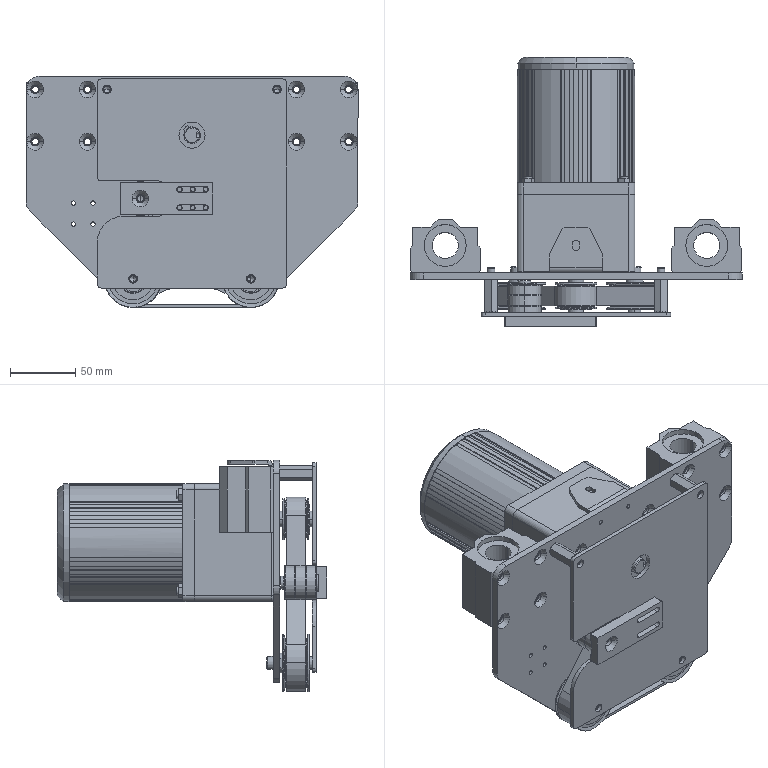Assembly | SolidWorks | mm | 19 component files | 21 solids | 2403 faces | box 254 x 206 x 177 mm | volume 1642860 mm3 | cylinder 1465 | plane 415 | cone 335 | torus 188 | commonest cylinder face diameters 0.56 x272 0.3 x253 3.95 x244 35.22 x82 37.44 x80 6.6 x38 25.67 x32 27.89 x31
Bill of materials:
BAY6000ZZ-J.stp | 3 | AISI 304 | Short thick annular ring with a central through bore; the face shows concentric outer ring, a recessed annular band, and an inner ring, like a shielded ball bearing seen from outside.
Belt11 | 1 |  | Thin-walled closed loop band of constant width. Its outline is a rounded, roughly triangular shape with an inward bend on one side.
EBF41-S3M150-30-A-N-d12.stp | 1 | 6061 Alloy | Toothed pulley-like cylinder with flanges at both ends and short hub bosses, a central bore with a keyway, and radial holes through the toothed rim.
EVD21-40-S3M150.stp | 2 | 6061 Alloy | Toothed pulley-like cylinder with flanges at both ends, a raised annular hub face on each side, and a plain central through bore with no keyway.
IK-AC(40W)InductionMotor[5IK40A1-C] | 1 |  | Square box-shaped block with rounded edges, joined coaxially to a longer cylindrical body that has lengthwise grooves and a chamfered far end. A single shaft sticks out of the square front face, off-centre, from a short stepped round boss. The overall form looks like a geared motor, but this is only a guess from the shape.
LMW01-d20.stp | 2 | 6061 Alloy | Prismatic housing block with a large through bore. The profile is stepped, with a raised top boss and stepped, chamfered lower shoulders. Four small holes are on one face, and there is an annular recess around the bore on the top face.
MDJ12-10-Y2-F23-E10-N6.stp | 2 | 45 | Stepped cylindrical pin. It has a long plain shank, a collar flange with two parallel flats, a narrow neck groove, and a short chamfered end section. An axial hole with a conical bottom is at one end.
MED02-10-Y2-F24.stp | 1 | 45 | Flanged cylindrical bushing/pin. It has a flange with two flats at one end, a long cylindrical body, a shallow circumferential groove near the opposite end, and an axial bore.
QX1-03-BJMotorMountingPlate | 1 | 201 Annealed Stainless Steel (SS) | Flat plate with a rectangular upper portion and tapered lower sides ending in a concave arc cutout. It has a large central round hole and many smaller holes, some with chamfered or countersunk edges.
QX1-08-BJAdapterBracket | 1 | Q235 | L-shaped bent plate bracket. One leg is tapered with a single elongated slot. The other leg is rectangular with two round holes. The two legs meet at a radiused bend.
QX1-23-BJCoverPlate | 1 | Q235 | Thin, nearly square flat plate with a rectangular notch cut into one side. It has a large round hole, a 2x3 grid of small holes, and four mounting holes near the corners.
QX1-24-TensionerSeat | 1 | 6061 Alloy | Rectangular bar with small chamfered corners. It has one countersunk through hole near one end and two parallel obround slots near the other end.
RBE12-S10-L25-M6-N6.stp | 2 |  | Hexagonal standoff-like part. It has a hex body with a female axial bore at one end, and a smaller cylindrical male stud with a relief neck and chamfered tip at the other.
Mates:
1. coincident | QX1-03-BJMotorMountingPlate-1 face at (52.203, 5.084, 478.747) dir (0, 1, 0) | IK-AC(40W)InductionMotor[5IK40A1-C]-1 face at (97.203, 5.084, 545.747) dir (0, -1, 0)
2. concentric | QX1-03-BJMotorMountingPlate-1 face at (52.203, 5.084, 518.747) dir (0, -1, 0) r 17.15 | IK-AC(40W)InductionMotor[5IK40A1-C]-1 face at (52.203, 5.084, 518.747) dir (0, 1, 0) r 6
3. parallel | QX1-03-BJMotorMountingPlate-1 face at (-74.797, 5.084, 563.747) dir (0, 0, 1) | IK-AC(40W)InductionMotor[5IK40A1-C]-1 face at (97.203, 65.084, 545.747) dir (0, 0, 1)
4. concentric | QX1-03-BJMotorMountingPlate-1 face at (7.203, 5.084, 408.747) dir (0, -1, 0) r 5.25 | EVD21-40-S3M150.stp-1 face at (7.203, -7.916, 408.747) dir (0, 1, 0) r 5
5. concentric | QX1-03-BJMotorMountingPlate-1 face at (97.203, 5.084, 408.747) dir (0, -1, 0) r 5.25 | EVD21-40-S3M150.stp-2 face at (97.203, -7.916, 408.747) dir (0, 1, 0) r 5
6. coincident | QX1-03-BJMotorMountingPlate-1 face at (52.203, 5.084, 478.747) dir (0, 1, 0) | LMW01-d20.stp-1 face at (-72.797, 5.084, 508.747) dir (0, -1, 0)
7. coincident | QX1-03-BJMotorMountingPlate-1 face at (52.203, 5.084, 478.747) dir (0, 1, 0) | LMW01-d20.stp-2 face at (162.703, 5.084, 508.747) dir (0, -1, 0)
8. coincident | QX1-03-BJMotorMountingPlate-1 face at (-74.797, 5.084, 393.747) dir (-1, 0, 0) | LMW01-d20.stp-1 face at (-74.797, 24.084, 508.747) dir (-1, 0, 0)
9. distance | QX1-03-BJMotorMountingPlate-1 face at (-74.797, 5.084, 563.747) dir (0, 0, 1) | LMW01-d20.stp-1 face at (-47.797, 26.084, 558.747) dir (0, 0, 1)
10. coincident | LMW01-d20.stp-2 face at (152.203, 26.084, 558.747) dir (0, 0, 1) | LMW01-d20.stp-1 face at (-47.797, 26.084, 558.747) dir (0, 0, 1)
11. parallel | LMW01-d20.stp-2 face at (162.703, 5.084, 508.747) dir (0, -1, 0) | LMW01-d20.stp-1 face at (-37.297, 5.084, 508.747) dir (0, -1, 0)
12. coincident | EVD21-40-S3M150.stp-1 face at (6.115, -22.916, 392.784) dir (0, -1, 0) | EVD21-40-S3M150.stp-2 face at (97.478, -22.916, 392.749) dir (0, -1, 0)
13. distance | EBF41-S3M150-30-A-N-d12.stp-1 face at (44.627, -1.916, 527.399) dir (0, 1, 0) | QX1-03-BJMotorMountingPlate-1 face at (52.203, 0.08384, 478.747) dir (0, -1, 0)
14. parallel | EBF41-S3M150-30-A-N-d12.stp-1 face at (42.687, -3.916, 529.614) dir (0, -1, 0) | EVD21-40-S3M150.stp-1 face at (6.115, -3.916, 392.784) dir (0, -1, 0)
15. coincident | EBF41-S3M150-30-A-N-d12.stp-1 face at (42.687, -3.916, 529.614) dir (0, -1, 0) | EVD21-40-S3M150.stp-1 face at (6.115, -3.916, 392.784) dir (0, -1, 0)
16. concentric | IK-AC(40W)InductionMotor[5IK40A1-C]-1 face at (52.203, 5.084, 518.747) dir (0, 1, 0) r 6 | EBF41-S3M150-30-A-N-d12.stp-1 face at (52.203, -1.916, 518.747) dir (0, -1, 0) r 6
17. coincident | QX1-03-BJMotorMountingPlate-1 face at (52.203, 5.084, 478.747) dir (0, 1, 0) | QX1-08-BJAdapterBracket-1 face at (32.203, 5.084, 548.747) dir (0, -1, 0)
18. coincident | QX1-03-BJMotorMountingPlate-1 face at (-74.797, 5.084, 563.747) dir (0, 0, 1) | QX1-08-BJAdapterBracket-1 face at (32.203, 5.084, 563.747) dir (0, 0, 1)
19. distance | QX1-08-BJAdapterBracket-1 face at (72.203, 8.084, 559.747) dir (1, 0, 0) | QX1-03-BJMotorMountingPlate-1 face at (179.203, 5.084, 393.747) dir (1, 0, 0)
20. concentric | EVD21-40-S3M150.stp-1 face at (7.203, -7.916, 408.747) dir (0, 1, 0) r 5 | QX1-23-BJCoverPlate-1 face at (7.203, -27.916, 408.747) dir (0, -1, 0) r 3.3
21. concentric | QX1-03-BJMotorMountingPlate-1 face at (-12.797, 0.08384, 553.747) dir (0, -1, 0) r 3.3 | QX1-23-BJCoverPlate-1 face at (-12.797, -27.916, 553.747) dir (0, -1, 0) r 3.3
22. concentric | Belt11-1 face at (52.203, -19.916, 518.747) dir (0, 1, 0) r 16.945 | IK-AC(40W)InductionMotor[5IK40A1-C]-1 face at (52.203, 5.084, 518.747) dir (0, 1, 0) r 6
23. concentric | Belt11-1 face at (7.203, -19.916, 408.747) dir (0, 1, 0) r 21.72 | EVD21-40-S3M150.stp-1 face at (7.203, -7.916, 408.747) dir (0, 1, 0) r 5
24. distance | Belt11-1 face at (52.203, -4.916, 518.747) dir (0, 1, 0) | EVD21-40-S3M150.stp-1 face at (6.115, -3.916, 392.784) dir (0, -1, 0)
25. distance | QX1-23-BJCoverPlate-1 face at (52.203, -24.916, 481.747) dir (0, 1, 0) | EVD21-40-S3M150.stp-1 face at (6.115, -22.916, 392.784) dir (0, -1, 0)
26. coincident | QX1-03-BJMotorMountingPlate-1 face at (52.203, 0.08384, 478.747) dir (0, -1, 0) | MDJ12-10-Y2-F23-E10-N6.stp-1 face at (7.203, 0.08384, 404.667) dir (0, 1, 0)
27. concentric | QX1-03-BJMotorMountingPlate-1 face at (7.203, 5.084, 408.747) dir (0, -1, 0) r 5.25 | MDJ12-10-Y2-F23-E10-N6.stp-1 face at (7.203, -24.916, 408.747) dir (0, 1, 0) r 5
28. coincident | QX1-03-BJMotorMountingPlate-1 face at (52.203, 0.08384, 478.747) dir (0, -1, 0) | MDJ12-10-Y2-F23-E10-N6.stp-2 face at (97.203, 0.08384, 404.667) dir (0, 1, 0)
29. concentric | QX1-03-BJMotorMountingPlate-1 face at (97.203, 5.084, 408.747) dir (0, -1, 0) r 5.25 | MDJ12-10-Y2-F23-E10-N6.stp-2 face at (97.203, -24.916, 408.747) dir (0, 1, 0) r 5
30. coincident | QX1-03-BJMotorMountingPlate-1 face at (52.203, 0.08384, 478.747) dir (0, -1, 0) | RBE12-S10-L25-M6-N6.stp-1 face at (-12.797, 0.08384, 553.747) dir (0, 1, 0)
31. concentric | QX1-03-BJMotorMountingPlate-1 face at (-12.797, 0.08384, 553.747) dir (0, -1, 0) r 3.3 | RBE12-S10-L25-M6-N6.stp-1 face at (-12.797, 0.08384, 553.747) dir (0, 1, 0) r 3
32. coincident | QX1-03-BJMotorMountingPlate-1 face at (52.203, 0.08384, 478.747) dir (0, -1, 0) | RBE12-S10-L25-M6-N6.stp-2 face at (117.203, 0.08384, 553.747) dir (0, 1, 0)
33. concentric | QX1-03-BJMotorMountingPlate-1 face at (117.203, 0.08384, 553.747) dir (0, -1, 0) r 3.3 | RBE12-S10-L25-M6-N6.stp-2 face at (117.203, 0.08384, 553.747) dir (0, 1, 0) r 3
34. coincident | QX1-23-BJCoverPlate-1 face at (52.203, -27.916, 481.747) dir (0, -1, 0) | QX1-24-TensionerSeat-1 face at (32.703, -27.916, 470.247) dir (0, 1, 0)
35. distance | QX1-23-BJCoverPlate-1 face at (-20.297, -24.916, 483.747) dir (0, 0, -1) | QX1-24-TensionerSeat-1 face at (67.703, -27.916, 482.747) dir (0, 0, 1)
36. coincident | QX1-24-TensionerSeat-1 face at (19.703, -29.916, 470.247) dir (0, 1, 0) | MED02-10-Y2-F24.stp-1 face at (15.703, -29.916, 470.247) dir (0, -1, 0)
37. concentric | QX1-24-TensionerSeat-1 face at (12.703, -35.916, 470.247) dir (0, -1, 0) r 3.3 | MED02-10-Y2-F24.stp-1 face at (12.703, -0.9162, 470.247) dir (0, -1, 0) r 5
38. parallel | QX1-24-TensionerSeat-1 face at (26.632, -29.916, 476.747) dir (0, 0, -1) | MED02-10-Y2-F24.stp-1 face at (5.203, -27.916, 476.747) dir (0, 0, 1)
39. concentric | MED02-10-Y2-F24.stp-1 face at (12.703, -0.9162, 470.247) dir (0, -1, 0) r 5 | BAY6000ZZ-J.stp-1 face at (12.703, -27.616, 470.247) dir (0, 1, 0) r 5
40. distance | QX1-23-BJCoverPlate-1 face at (-20.297, -24.916, 401.747) dir (-1, 0, 0) | QX1-24-TensionerSeat-1 face at (-2.297, -27.916, 457.747) dir (-1, 0, 0)